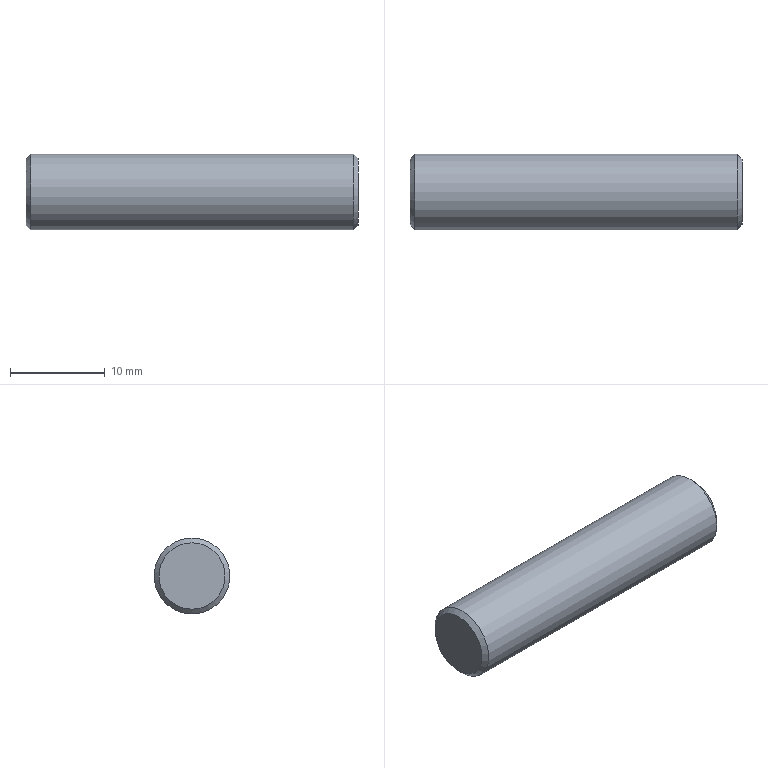Component | NX | LARGE_PIN_2 | 1 solid | 5 faces | box 35 x 8 x 8 mm | volume 1753 mm3 | plane 2 | cone 2 | cylinder 1 | commonest cylinder face diameters 8 x1
STEP:
#1=CARTESIAN_POINT('',(0.,0.,0.));
#2=DIRECTION('',(0.,0.,1.));
#3=DIRECTION('',(1.,0.,0.));
#4=AXIS2_PLACEMENT_3D('',#1,#2,#3);
#5=CARTESIAN_POINT('',(12.495,128.395,125.614));
#6=VERTEX_POINT('',#5);
#7=CARTESIAN_POINT('',(12.495,128.395,129.114));
#8=DIRECTION('',(1.,0.,0.));
#9=DIRECTION('',(0.,0.,-1.));
#10=AXIS2_PLACEMENT_3D('',#7,#8,#9);
#11=CIRCLE('',#10,3.5);
#12=CARTESIAN_POINT('',(12.495,128.395,129.114));
#13=DIRECTION('',(1.,0.,0.));
#14=DIRECTION('',(0.,0.,-1.));
#15=AXIS2_PLACEMENT_3D('',#12,#13,#14);
#16=PLANE('',#15);
#17=CARTESIAN_POINT('',(0.,0.));
#18=DIRECTION('',(1.,0.));
#19=AXIS2_PLACEMENT_2D('',#17,#18);
#20=CIRCLE('',#19,3.5);
#21=(GEOMETRIC_REPRESENTATION_CONTEXT(2)PARAMETRIC_REPRESENTATION_CONTEXT()REPRESENTATION_CONTEXT('',''));
#22=DEFINITIONAL_REPRESENTATION('',(#20),#21);
#23=PCURVE('',#16,#22);
#24=CARTESIAN_POINT('',(11.995,128.395,129.114));
#25=DIRECTION('',(-1.,0.,0.));
#26=DIRECTION('',(0.,0.,1.));
#27=AXIS2_PLACEMENT_3D('',#24,#25,#26);
#28=CONICAL_SURFACE('',#27,4.,0.7854);
#29=CARTESIAN_POINT('',(9.425,-0.5));
#30=DIRECTION('',(-1.,0.));
#31=VECTOR('',#30,1.);
#32=LINE('',#29,#31);
#33=(GEOMETRIC_REPRESENTATION_CONTEXT(2)PARAMETRIC_REPRESENTATION_CONTEXT()REPRESENTATION_CONTEXT('',''));
#34=DEFINITIONAL_REPRESENTATION('',(#32),#33);
#35=PCURVE('',#28,#34);
#36=SURFACE_CURVE('',#11,(#23,#35),.PCURVE_S1.);
#37=EDGE_CURVE('',#6,#6,#36,.T.);
#38=ORIENTED_EDGE('',*,*,#37,.T.);
#39=EDGE_LOOP('',(#38));
#40=FACE_BOUND('',#39,.T.);
#41=ADVANCED_FACE('',(#40),#16,.T.);
#42=CARTESIAN_POINT('',(-22.505,128.395,132.614));
#43=VERTEX_POINT('',#42);
#44=CARTESIAN_POINT('',(-22.505,128.395,129.114));
#45=DIRECTION('',(-1.,0.,0.));
#46=DIRECTION('',(0.,0.,1.));
#47=AXIS2_PLACEMENT_3D('',#44,#45,#46);
#48=CIRCLE('',#47,3.5);
#49=CARTESIAN_POINT('',(-22.505,128.395,129.114));
#50=DIRECTION('',(-1.,0.,0.));
#51=DIRECTION('',(0.,0.,1.));
#52=AXIS2_PLACEMENT_3D('',#49,#50,#51);
#53=PLANE('',#52);
#54=CARTESIAN_POINT('',(0.,0.));
#55=DIRECTION('',(1.,0.));
#56=AXIS2_PLACEMENT_2D('',#54,#55);
#57=CIRCLE('',#56,3.5);
#58=(GEOMETRIC_REPRESENTATION_CONTEXT(2)PARAMETRIC_REPRESENTATION_CONTEXT()REPRESENTATION_CONTEXT('',''));
#59=DEFINITIONAL_REPRESENTATION('',(#57),#58);
#60=PCURVE('',#53,#59);
#61=CARTESIAN_POINT('',(-22.005,128.395,129.114));
#62=DIRECTION('',(1.,0.,0.));
#63=DIRECTION('',(0.,0.,-1.));
#64=AXIS2_PLACEMENT_3D('',#61,#62,#63);
#65=CONICAL_SURFACE('',#64,4.,0.7854);
#66=CARTESIAN_POINT('',(9.425,-0.5));
#67=DIRECTION('',(-1.,0.));
#68=VECTOR('',#67,1.);
#69=LINE('',#66,#68);
#70=(GEOMETRIC_REPRESENTATION_CONTEXT(2)PARAMETRIC_REPRESENTATION_CONTEXT()REPRESENTATION_CONTEXT('',''));
#71=DEFINITIONAL_REPRESENTATION('',(#69),#70);
#72=PCURVE('',#65,#71);
#73=SURFACE_CURVE('',#48,(#60,#72),.PCURVE_S1.);
#74=EDGE_CURVE('',#43,#43,#73,.T.);
#75=ORIENTED_EDGE('',*,*,#74,.T.);
#76=EDGE_LOOP('',(#75));
#77=FACE_BOUND('',#76,.T.);
#78=ADVANCED_FACE('',(#77),#53,.T.);
#79=CARTESIAN_POINT('',(-22.005,128.395,133.114));
#80=VERTEX_POINT('',#79);
#81=CARTESIAN_POINT('',(-22.005,128.395,125.114));
#82=VERTEX_POINT('',#81);
#83=CARTESIAN_POINT('',(-22.005,128.395,129.114));
#84=DIRECTION('',(1.,0.,0.));
#85=DIRECTION('',(0.,0.,1.));
#86=AXIS2_PLACEMENT_3D('',#83,#84,#85);
#87=CIRCLE('',#86,4.);
#88=CARTESIAN_POINT('',(-22.505,128.395,129.114));
#89=DIRECTION('',(1.,0.,0.));
#90=DIRECTION('',(0.,0.,-1.));
#91=AXIS2_PLACEMENT_3D('',#88,#89,#90);
#92=CYLINDRICAL_SURFACE('',#91,4.);
#93=CARTESIAN_POINT('',(3.142,0.5));
#94=DIRECTION('',(1.,0.));
#95=VECTOR('',#94,1.);
#96=LINE('',#93,#95);
#97=(GEOMETRIC_REPRESENTATION_CONTEXT(2)PARAMETRIC_REPRESENTATION_CONTEXT()REPRESENTATION_CONTEXT('',''));
#98=DEFINITIONAL_REPRESENTATION('',(#96),#97);
#99=PCURVE('',#92,#98);
#100=CARTESIAN_POINT('',(3.142,0.));
#101=DIRECTION('',(1.,0.));
#102=VECTOR('',#101,1.);
#103=LINE('',#100,#102);
#104=(GEOMETRIC_REPRESENTATION_CONTEXT(2)PARAMETRIC_REPRESENTATION_CONTEXT()REPRESENTATION_CONTEXT('',''));
#105=DEFINITIONAL_REPRESENTATION('',(#103),#104);
#106=PCURVE('',#65,#105);
#107=SURFACE_CURVE('',#87,(#99,#106),.PCURVE_S1.);
#108=EDGE_CURVE('',#80,#82,#107,.T.);
#109=ORIENTED_EDGE('',*,*,#108,.T.);
#110=CARTESIAN_POINT('',(11.995,128.395,125.114));
#111=VERTEX_POINT('',#110);
#112=CARTESIAN_POINT('',(-22.005,128.395,125.114));
#113=CARTESIAN_POINT('',(11.995,128.395,125.114));
#114=B_SPLINE_CURVE_WITH_KNOTS('',1,(#112,#113),.UNSPECIFIED.,.F.,.F.,(2,2),(0.5,34.5),.PIECEWISE_BEZIER_KNOTS.);
#115=CARTESIAN_POINT('',(6.283,0.));
#116=DIRECTION('',(0.,1.));
#117=VECTOR('',#116,1.);
#118=LINE('',#115,#117);
#119=(GEOMETRIC_REPRESENTATION_CONTEXT(2)PARAMETRIC_REPRESENTATION_CONTEXT()REPRESENTATION_CONTEXT('',''));
#120=DEFINITIONAL_REPRESENTATION('',(#118),#119);
#121=PCURVE('',#92,#120);
#122=CARTESIAN_POINT('',(0.,0.));
#123=DIRECTION('',(0.,1.));
#124=VECTOR('',#123,1.);
#125=LINE('',#122,#124);
#126=(GEOMETRIC_REPRESENTATION_CONTEXT(2)PARAMETRIC_REPRESENTATION_CONTEXT()REPRESENTATION_CONTEXT('',''));
#127=DEFINITIONAL_REPRESENTATION('',(#125),#126);
#128=PCURVE('',#92,#127);
#129=SEAM_CURVE('',#114,(#121,#128),.PCURVE_S1.);
#130=EDGE_CURVE('',#82,#111,#129,.T.);
#131=ORIENTED_EDGE('',*,*,#130,.T.);
#132=CARTESIAN_POINT('',(11.995,128.395,129.114));
#133=DIRECTION('',(-1.,0.,0.));
#134=DIRECTION('',(0.,0.,-1.));
#135=AXIS2_PLACEMENT_3D('',#132,#133,#134);
#136=CIRCLE('',#135,4.);
#137=CARTESIAN_POINT('',(6.283,34.5));
#138=DIRECTION('',(-1.,0.));
#139=VECTOR('',#138,1.);
#140=LINE('',#137,#139);
#141=(GEOMETRIC_REPRESENTATION_CONTEXT(2)PARAMETRIC_REPRESENTATION_CONTEXT()REPRESENTATION_CONTEXT('',''));
#142=DEFINITIONAL_REPRESENTATION('',(#140),#141);
#143=PCURVE('',#92,#142);
#144=CARTESIAN_POINT('',(3.142,0.));
#145=DIRECTION('',(1.,0.));
#146=VECTOR('',#145,1.);
#147=LINE('',#144,#146);
#148=(GEOMETRIC_REPRESENTATION_CONTEXT(2)PARAMETRIC_REPRESENTATION_CONTEXT()REPRESENTATION_CONTEXT('',''));
#149=DEFINITIONAL_REPRESENTATION('',(#147),#148);
#150=PCURVE('',#28,#149);
#151=SURFACE_CURVE('',#136,(#143,#150),.PCURVE_S1.);
#152=EDGE_CURVE('',#111,#111,#151,.T.);
#153=ORIENTED_EDGE('',*,*,#152,.T.);
#154=ORIENTED_EDGE('',*,*,#130,.F.);
#155=CARTESIAN_POINT('',(-22.005,128.395,129.114));
#156=DIRECTION('',(1.,0.,0.));
#157=DIRECTION('',(0.,0.,1.));
#158=AXIS2_PLACEMENT_3D('',#155,#156,#157);
#159=CIRCLE('',#158,4.);
#160=CARTESIAN_POINT('',(-3.142,0.5));
#161=DIRECTION('',(1.,0.));
#162=VECTOR('',#161,1.);
#163=LINE('',#160,#162);
#164=(GEOMETRIC_REPRESENTATION_CONTEXT(2)PARAMETRIC_REPRESENTATION_CONTEXT()REPRESENTATION_CONTEXT('',''));
#165=DEFINITIONAL_REPRESENTATION('',(#163),#164);
#166=PCURVE('',#92,#165);
#167=CARTESIAN_POINT('',(3.142,0.));
#168=DIRECTION('',(1.,0.));
#169=VECTOR('',#168,1.);
#170=LINE('',#167,#169);
#171=(GEOMETRIC_REPRESENTATION_CONTEXT(2)PARAMETRIC_REPRESENTATION_CONTEXT()REPRESENTATION_CONTEXT('',''));
#172=DEFINITIONAL_REPRESENTATION('',(#170),#171);
#173=PCURVE('',#65,#172);
#174=SURFACE_CURVE('',#159,(#166,#173),.PCURVE_S1.);
#175=EDGE_CURVE('',#82,#80,#174,.T.);
#176=ORIENTED_EDGE('',*,*,#175,.T.);
#177=EDGE_LOOP('',(#109,#131,#153,#154,#176));
#178=FACE_BOUND('',#177,.T.);
#179=ADVANCED_FACE('',(#178),#92,.T.);
#180=ORIENTED_EDGE('',*,*,#74,.F.);
#181=CARTESIAN_POINT('',(-22.505,128.395,132.614));
#182=CARTESIAN_POINT('',(-22.005,128.395,133.114));
#183=B_SPLINE_CURVE_WITH_KNOTS('',1,(#181,#182),.UNSPECIFIED.,.F.,.F.,(2,2),(-0.7071,0.),.PIECEWISE_BEZIER_KNOTS.);
#184=CARTESIAN_POINT('',(9.425,0.));
#185=DIRECTION('',(0.,1.));
#186=VECTOR('',#185,1.);
#187=LINE('',#184,#186);
#188=(GEOMETRIC_REPRESENTATION_CONTEXT(2)PARAMETRIC_REPRESENTATION_CONTEXT()REPRESENTATION_CONTEXT('',''));
#189=DEFINITIONAL_REPRESENTATION('',(#187),#188);
#190=PCURVE('',#65,#189);
#191=CARTESIAN_POINT('',(3.142,0.));
#192=DIRECTION('',(0.,1.));
#193=VECTOR('',#192,1.);
#194=LINE('',#191,#193);
#195=(GEOMETRIC_REPRESENTATION_CONTEXT(2)PARAMETRIC_REPRESENTATION_CONTEXT()REPRESENTATION_CONTEXT('',''));
#196=DEFINITIONAL_REPRESENTATION('',(#194),#195);
#197=PCURVE('',#65,#196);
#198=SEAM_CURVE('',#183,(#190,#197),.PCURVE_S1.);
#199=EDGE_CURVE('',#43,#80,#198,.T.);
#200=ORIENTED_EDGE('',*,*,#199,.T.);
#201=ORIENTED_EDGE('',*,*,#175,.F.);
#202=ORIENTED_EDGE('',*,*,#108,.F.);
#203=ORIENTED_EDGE('',*,*,#199,.F.);
#204=EDGE_LOOP('',(#180,#200,#201,#202,#203));
#205=FACE_BOUND('',#204,.T.);
#206=ADVANCED_FACE('',(#205),#65,.T.);
#207=ORIENTED_EDGE('',*,*,#37,.F.);
#208=CARTESIAN_POINT('',(12.495,128.395,125.614));
#209=CARTESIAN_POINT('',(11.995,128.395,125.114));
#210=B_SPLINE_CURVE_WITH_KNOTS('',1,(#208,#209),.UNSPECIFIED.,.F.,.F.,(2,2),(-0.7071,0.),.PIECEWISE_BEZIER_KNOTS.);
#211=CARTESIAN_POINT('',(9.425,0.));
#212=DIRECTION('',(0.,1.));
#213=VECTOR('',#212,1.);
#214=LINE('',#211,#213);
#215=(GEOMETRIC_REPRESENTATION_CONTEXT(2)PARAMETRIC_REPRESENTATION_CONTEXT()REPRESENTATION_CONTEXT('',''));
#216=DEFINITIONAL_REPRESENTATION('',(#214),#215);
#217=PCURVE('',#28,#216);
#218=CARTESIAN_POINT('',(3.142,0.));
#219=DIRECTION('',(0.,1.));
#220=VECTOR('',#219,1.);
#221=LINE('',#218,#220);
#222=(GEOMETRIC_REPRESENTATION_CONTEXT(2)PARAMETRIC_REPRESENTATION_CONTEXT()REPRESENTATION_CONTEXT('',''));
#223=DEFINITIONAL_REPRESENTATION('',(#221),#222);
#224=PCURVE('',#28,#223);
#225=SEAM_CURVE('',#210,(#217,#224),.PCURVE_S1.);
#226=EDGE_CURVE('',#6,#111,#225,.T.);
#227=ORIENTED_EDGE('',*,*,#226,.T.);
#228=ORIENTED_EDGE('',*,*,#152,.F.);
#229=ORIENTED_EDGE('',*,*,#226,.F.);
#230=EDGE_LOOP('',(#207,#227,#228,#229));
#231=FACE_BOUND('',#230,.T.);
#232=ADVANCED_FACE('',(#231),#28,.T.);
#233=CLOSED_SHELL('',(#41,#78,#179,#206,#232));
#234=MANIFOLD_SOLID_BREP('',#233);
#235=(LENGTH_UNIT()NAMED_UNIT(*)SI_UNIT(.MILLI.,.METRE.));
#236=UNCERTAINTY_MEASURE_WITH_UNIT(LENGTH_MEASURE(0.00001),#235,'','');
#237=(NAMED_UNIT(*)PLANE_ANGLE_UNIT()SI_UNIT($,.RADIAN.));
#238=(NAMED_UNIT(*)SI_UNIT($,.STERADIAN.)SOLID_ANGLE_UNIT());
#239=(GEOMETRIC_REPRESENTATION_CONTEXT(3)GLOBAL_UNCERTAINTY_ASSIGNED_CONTEXT((#236))GLOBAL_UNIT_ASSIGNED_CONTEXT((#235,#237,#238))REPRESENTATION_CONTEXT('',''));
#240=ADVANCED_BREP_SHAPE_REPRESENTATION('',(#4,#234),#239);